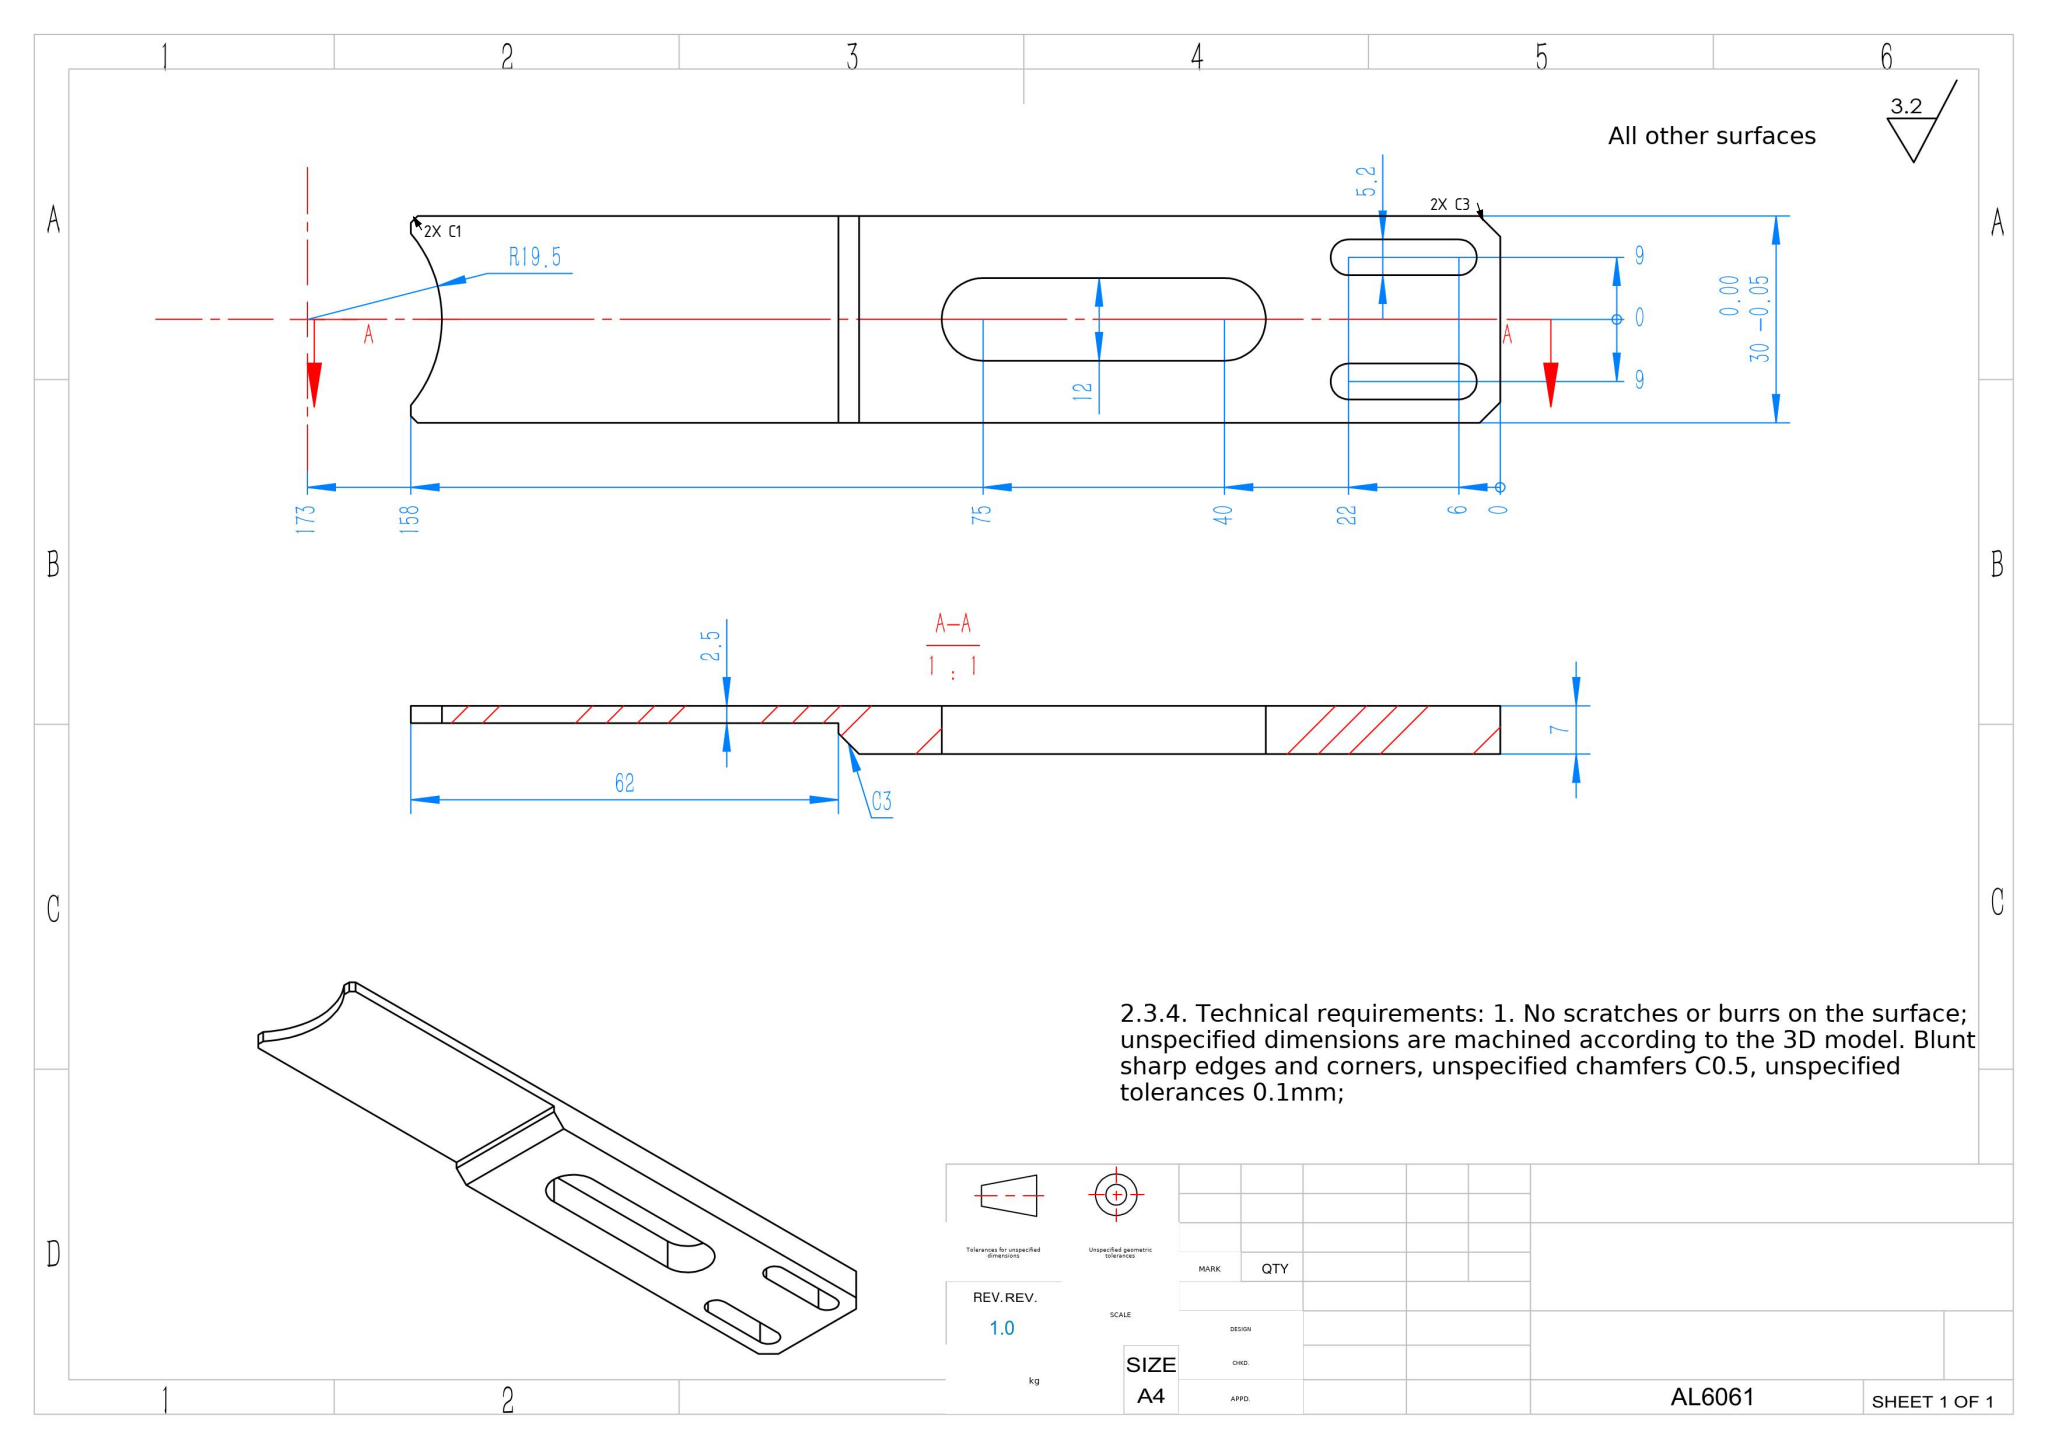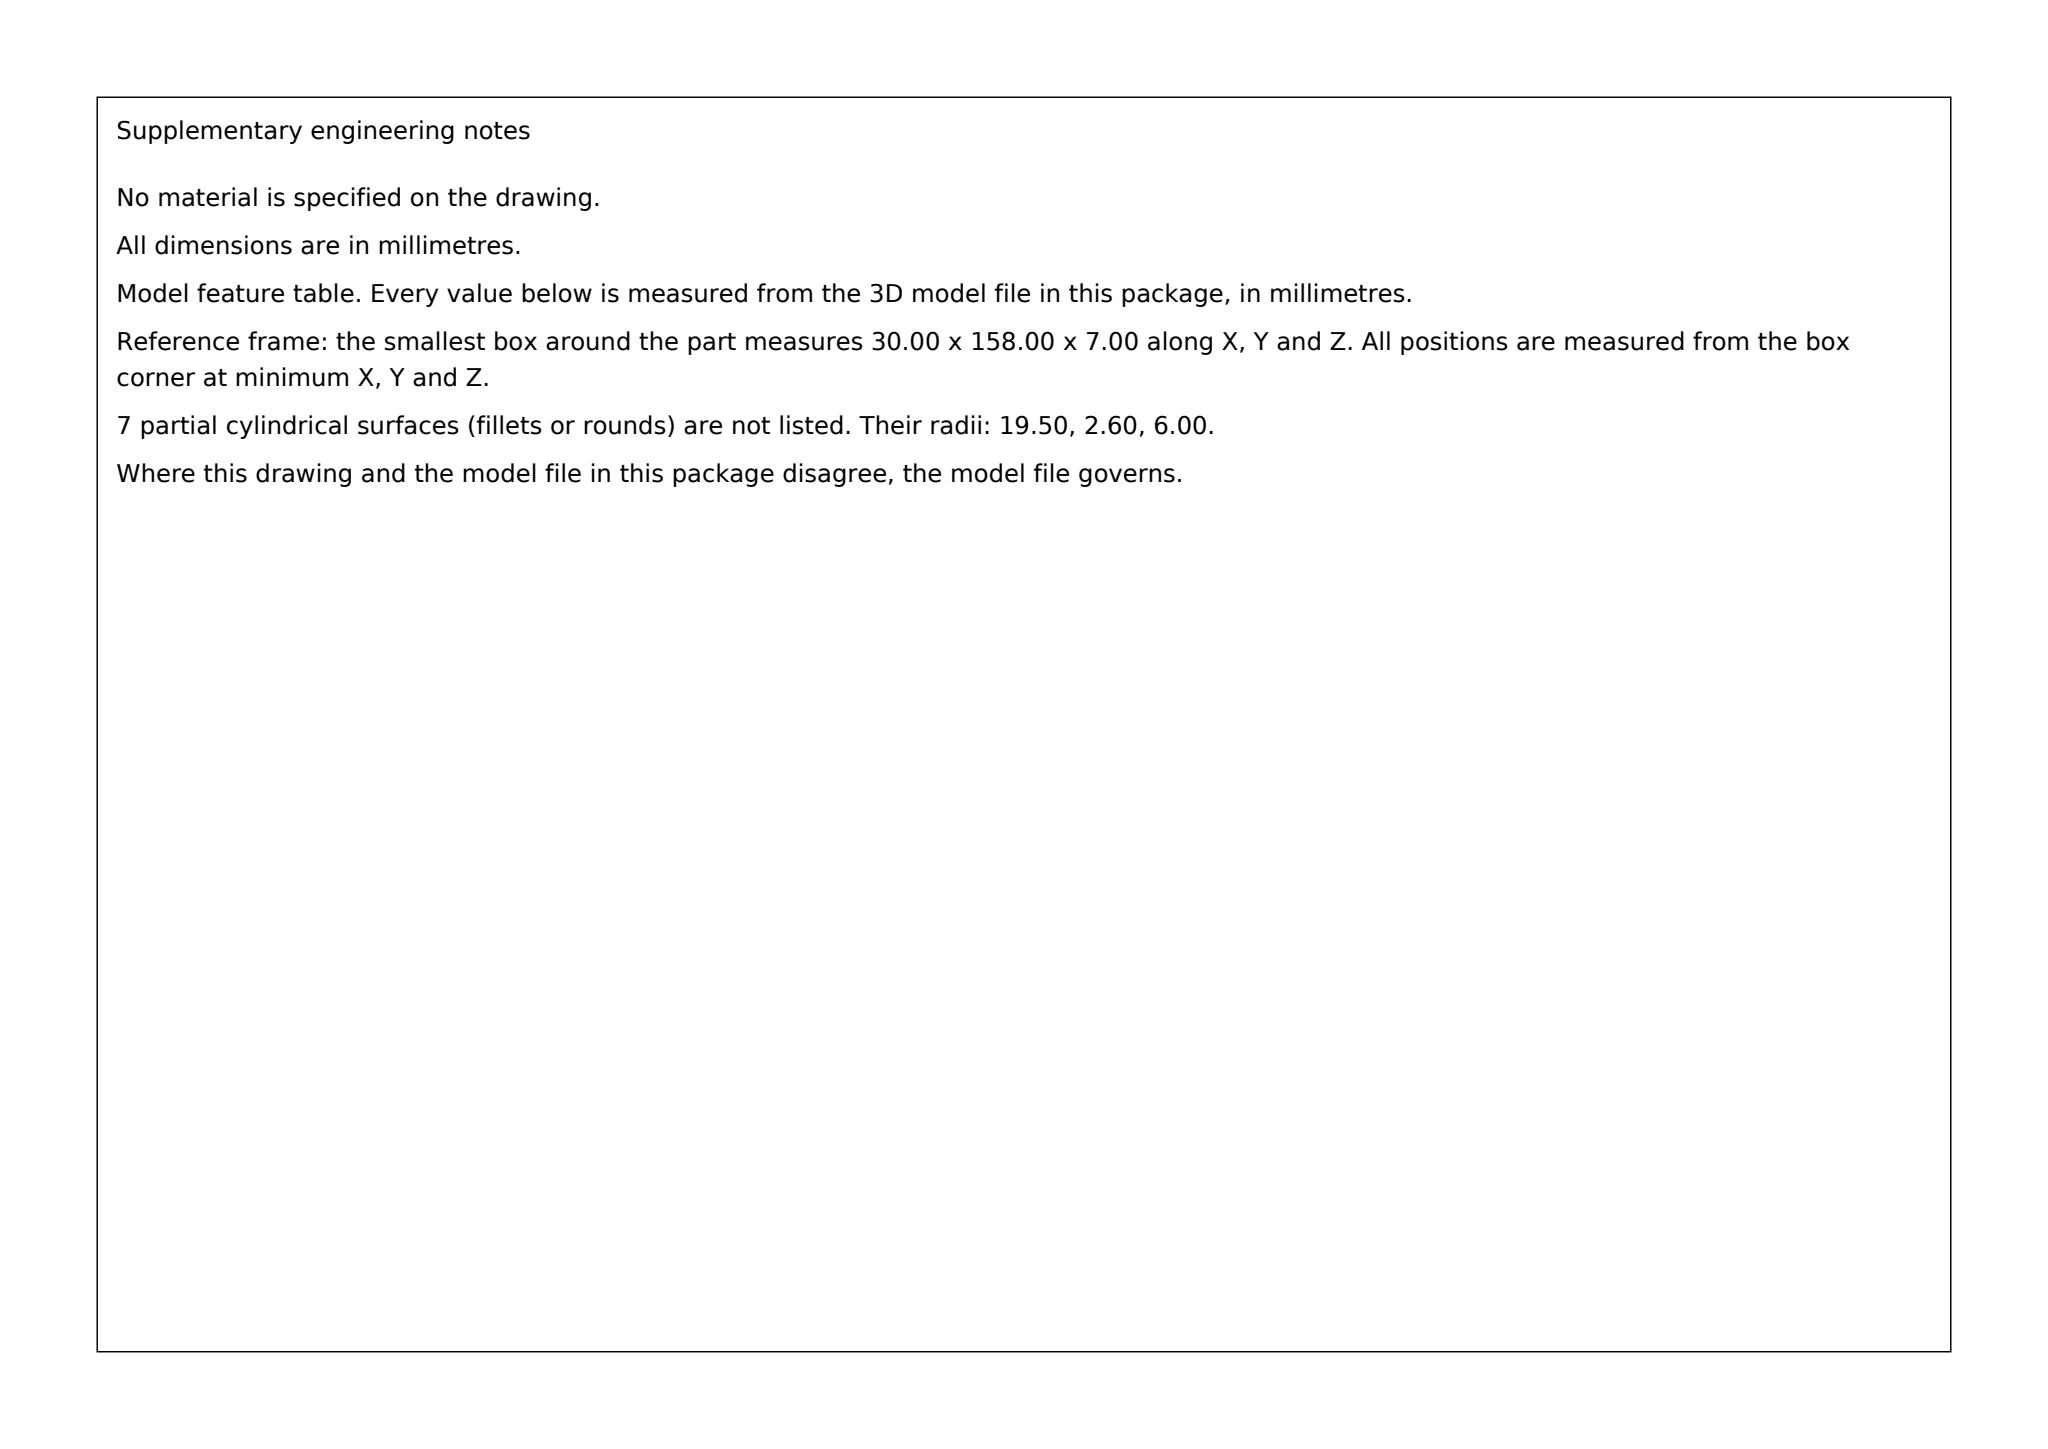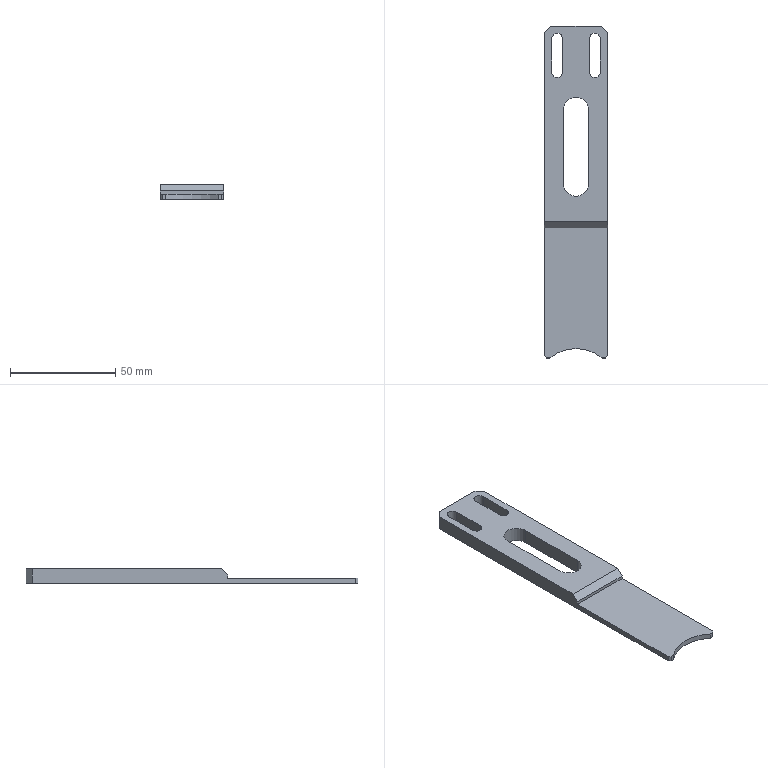Part | SolidWorks | mm | material AL6061 | 1 solid | 27 faces | box 30 x 158 x 7 mm | volume 19224 mm3 | plane 20 | cylinder 7 | commonest cylinder face diameters 5.2 x4 12 x2 39 x1
Drawing notes:
2X CHAMFER 3 X 45° ON THE TWO CORNERS OF THE 30 WIDE END FACE AT THE 0 DATUM END (158 FROM THE RADIUSED END), FULL 7 THICKNESS | from the solid: inclined_planes: two 45/45/90 faces, bbox_from [0,155,0] and [27,155,0], size [3,3,7]; y=158 end face extent x 3..27
2X CHAMFER 1 X 45° ON THE TWO CORNERS OF THE OPPOSITE (RADIUSED, 173 DATUM) END, WITHIN THE 2.5 THICK STEP | from the solid: inclined_planes: two 45/45/90 faces, bbox_from [0,0,0] and [29,0,0], size [1,1,2.5]
build123d program:
from build123d import *

# Parameters (mm, degrees)
SKETCH1_W               = 30
SKETCH1_H               = 158
BOSS_EXTRUDE1_DEPTH     = 1.25
SKETCH3_W               = 30
SKETCH3_H               = 96
BOSS_EXTRUDE2_DEPTH     = 4.5
CUT_EXTRUDE1_DEPTH      = 81.537
CUT_EXTRUDE1_DEPTH_BACK = 81.537
SKETCH2_R               = 19.5
CUT_EXTRUDE2_DEPTH      = 81.716
CHAMFER1_SIZE           = 3
CUT_EXTRUDE3_DEPTH      = 81.716
CHAMFER2_SIZE           = 3
CHAMFER4_SIZE           = 1


with BuildPart() as part:
    # Sketch1 → Boss-Extrude1 (new, symmetric)
    with BuildSketch(Plane.XY):
        Rectangle(SKETCH1_W, SKETCH1_H)
    extrude(amount=BOSS_EXTRUDE1_DEPTH, both=True)

    # Sketch3 → Boss-Extrude2 (add)
    with BuildSketch(Plane.XY.offset(1.25)):
        with Locations((0, 31)):
            Rectangle(SKETCH3_W, SKETCH3_H)
    extrude(amount=BOSS_EXTRUDE2_DEPTH)

    # Sketch2 → Cut-Extrude1 (cut, two sides: drawn at the far end of the back side and taken through both)
    with BuildSketch(Plane.XY.offset(1.25).offset(-CUT_EXTRUDE1_DEPTH_BACK)):
        with Locations((0, -94)):
            Circle(SKETCH2_R)
    extrude(amount=CUT_EXTRUDE1_DEPTH + CUT_EXTRUDE1_DEPTH_BACK, mode=Mode.SUBTRACT)

    # Sketch4 → Cut-Extrude2 (cut, through all)
    with BuildSketch(Plane.XY.offset(5.75)):
        with BuildLine():
            Line((-11.6, 57), (-11.6, 73))
            ThreePointArc((-11.6, 73), (-9, 75.6), (-6.4, 73))
            Line((-6.4, 73), (-6.4, 57))
            ThreePointArc((-6.4, 57), (-9, 54.4), (-11.6, 57))
        make_face()
        with BuildLine():
            Line((6.4, 57), (6.4, 73))
            ThreePointArc((6.4, 73), (9, 75.6), (11.6, 73))
            Line((11.6, 73), (11.6, 57))
            ThreePointArc((11.6, 57), (9, 54.4), (6.4, 57))
        make_face()
    extrude(amount=-CUT_EXTRUDE2_DEPTH, mode=Mode.SUBTRACT)

    # Chamfer1
    chamfer1_edges = [part.edges().sort_by_distance(p)[0] for p in [
        (0, -17, 5.75),
    ]]
    chamfer(chamfer1_edges, length=CHAMFER1_SIZE)

    # Sketch5 → Cut-Extrude3 (cut, through all)
    with BuildSketch(Plane.XY.offset(5.75)):
        with BuildLine():
            Line((-6, 4), (-6, 39))
            ThreePointArc((-6, 39), (0, 45), (6, 39))
            Line((6, 39), (6, 4))
            ThreePointArc((6, 4), (0, -2), (-6, 4))
        make_face()
    extrude(amount=-CUT_EXTRUDE3_DEPTH, mode=Mode.SUBTRACT)

    # Chamfer2
    chamfer2_edges = [part.edges().sort_by_distance(p)[0] for p in [
        (-15, 79, 2.25),
        (15, 79, 2.25),
    ]]
    chamfer(chamfer2_edges, length=CHAMFER2_SIZE)

    # Chamfer4
    chamfer4_edges = [part.edges().sort_by_distance(p)[0] for p in [
        (15, -79, 0),
        (-15, -79, 0),
    ]]
    chamfer(chamfer4_edges, length=CHAMFER4_SIZE)


solid = part.part
STEP:
#1=CARTESIAN_POINT('',(-14.,-79.,1.25));
#2=VERTEX_POINT('',#1);
#3=CARTESIAN_POINT('',(-12.46,-79.,1.25));
#4=VERTEX_POINT('',#3);
#5=CARTESIAN_POINT('',(-15.,-79.,1.25));
#6=DIRECTION('',(1.,0.,0.));
#7=VECTOR('',#6,1000.);
#8=LINE('',#5,#7);
#9=EDGE_CURVE('',#2,#4,#8,.T.);
#10=ORIENTED_EDGE('',*,*,#9,.F.);
#11=CARTESIAN_POINT('',(-14.,-79.,-1.25));
#12=VERTEX_POINT('',#11);
#13=CARTESIAN_POINT('',(-14.,-79.,1.25));
#14=DIRECTION('',(0.,0.,-1.));
#15=VECTOR('',#14,1000.);
#16=LINE('',#13,#15);
#17=EDGE_CURVE('',#2,#12,#16,.T.);
#18=ORIENTED_EDGE('',*,*,#17,.T.);
#19=CARTESIAN_POINT('',(-12.46,-79.,-1.25));
#20=VERTEX_POINT('',#19);
#21=CARTESIAN_POINT('',(-15.,-79.,-1.25));
#22=DIRECTION('',(1.,0.,0.));
#23=VECTOR('',#22,1000.);
#24=LINE('',#21,#23);
#25=EDGE_CURVE('',#12,#20,#24,.T.);
#26=ORIENTED_EDGE('',*,*,#25,.T.);
#27=CARTESIAN_POINT('',(-12.46,-79.,-1.25));
#28=DIRECTION('',(0.,0.,1.));
#29=VECTOR('',#28,1000.);
#30=LINE('',#27,#29);
#31=EDGE_CURVE('',#20,#4,#30,.T.);
#32=ORIENTED_EDGE('',*,*,#31,.T.);
#33=EDGE_LOOP('',(#10,#18,#26,#32));
#34=FACE_OUTER_BOUND('',#33,.T.);
#35=CARTESIAN_POINT('',(-15.,-79.,1.25));
#36=DIRECTION('',(0.,1.,0.));
#37=DIRECTION('',(0.,0.,1.));
#38=AXIS2_PLACEMENT_3D('',#35,#36,#37);
#39=PLANE('',#38);
#40=ADVANCED_FACE('',(#34),#39,.F.);
#41=CARTESIAN_POINT('',(-15.,-17.,1.25));
#42=VERTEX_POINT('',#41);
#43=CARTESIAN_POINT('',(-15.,-78.,1.25));
#44=VERTEX_POINT('',#43);
#45=CARTESIAN_POINT('',(-15.,-79.,1.25));
#46=DIRECTION('',(0.,-1.,0.));
#47=VECTOR('',#46,1000.);
#48=LINE('',#45,#47);
#49=EDGE_CURVE('',#42,#44,#48,.T.);
#50=ORIENTED_EDGE('',*,*,#49,.T.);
#51=CARTESIAN_POINT('',(-14.,-79.,1.25));
#52=DIRECTION('',(0.7071,-0.7071,0.));
#53=VECTOR('',#52,1000.);
#54=LINE('',#51,#53);
#55=EDGE_CURVE('',#44,#2,#54,.T.);
#56=ORIENTED_EDGE('',*,*,#55,.T.);
#57=ORIENTED_EDGE('',*,*,#9,.T.);
#58=CARTESIAN_POINT('',(12.46,-79.,1.25));
#59=VERTEX_POINT('',#58);
#60=CARTESIAN_POINT('',(0.,-94.,1.25));
#61=DIRECTION('',(0.,0.,-1.));
#62=DIRECTION('',(-1.,0.,0.));
#63=AXIS2_PLACEMENT_3D('',#60,#61,#62);
#64=CIRCLE('',#63,19.5);
#65=EDGE_CURVE('',#4,#59,#64,.T.);
#66=ORIENTED_EDGE('',*,*,#65,.T.);
#67=CARTESIAN_POINT('',(14.,-79.,1.25));
#68=VERTEX_POINT('',#67);
#69=CARTESIAN_POINT('',(-15.,-79.,1.25));
#70=DIRECTION('',(1.,0.,0.));
#71=VECTOR('',#70,1000.);
#72=LINE('',#69,#71);
#73=EDGE_CURVE('',#59,#68,#72,.T.);
#74=ORIENTED_EDGE('',*,*,#73,.T.);
#75=CARTESIAN_POINT('',(15.,-78.,1.25));
#76=VERTEX_POINT('',#75);
#77=CARTESIAN_POINT('',(15.,-78.,1.25));
#78=DIRECTION('',(0.7071,0.7071,0.));
#79=VECTOR('',#78,1000.);
#80=LINE('',#77,#79);
#81=EDGE_CURVE('',#68,#76,#80,.T.);
#82=ORIENTED_EDGE('',*,*,#81,.T.);
#83=CARTESIAN_POINT('',(15.,-17.,1.25));
#84=VERTEX_POINT('',#83);
#85=CARTESIAN_POINT('',(15.,-79.,1.25));
#86=DIRECTION('',(0.,1.,0.));
#87=VECTOR('',#86,1000.);
#88=LINE('',#85,#87);
#89=EDGE_CURVE('',#76,#84,#88,.T.);
#90=ORIENTED_EDGE('',*,*,#89,.T.);
#91=CARTESIAN_POINT('',(-15.,-17.,1.25));
#92=DIRECTION('',(1.,0.,0.));
#93=VECTOR('',#92,1000.);
#94=LINE('',#91,#93);
#95=EDGE_CURVE('',#42,#84,#94,.T.);
#96=ORIENTED_EDGE('',*,*,#95,.F.);
#97=EDGE_LOOP('',(#50,#56,#57,#66,#74,#82,#90,#96));
#98=FACE_OUTER_BOUND('',#97,.T.);
#99=CARTESIAN_POINT('',(0.,0.,1.25));
#100=DIRECTION('',(0.,0.,-1.));
#101=DIRECTION('',(-1.,0.,0.));
#102=AXIS2_PLACEMENT_3D('',#99,#100,#101);
#103=PLANE('',#102);
#104=ADVANCED_FACE('',(#98),#103,.F.);
#105=ORIENTED_EDGE('',*,*,#89,.F.);
#106=CARTESIAN_POINT('',(15.,-78.,-1.25));
#107=VERTEX_POINT('',#106);
#108=CARTESIAN_POINT('',(15.,-78.,1.25));
#109=DIRECTION('',(0.,0.,-1.));
#110=VECTOR('',#109,1000.);
#111=LINE('',#108,#110);
#112=EDGE_CURVE('',#76,#107,#111,.T.);
#113=ORIENTED_EDGE('',*,*,#112,.T.);
#114=CARTESIAN_POINT('',(15.,76.,-1.25));
#115=VERTEX_POINT('',#114);
#116=CARTESIAN_POINT('',(15.,-79.,-1.25));
#117=DIRECTION('',(0.,1.,0.));
#118=VECTOR('',#117,1000.);
#119=LINE('',#116,#118);
#120=EDGE_CURVE('',#107,#115,#119,.T.);
#121=ORIENTED_EDGE('',*,*,#120,.T.);
#122=CARTESIAN_POINT('',(15.,76.,5.75));
#123=VERTEX_POINT('',#122);
#124=CARTESIAN_POINT('',(15.,76.,1.25));
#125=DIRECTION('',(0.,0.,1.));
#126=VECTOR('',#125,1000.);
#127=LINE('',#124,#126);
#128=EDGE_CURVE('',#115,#123,#127,.T.);
#129=ORIENTED_EDGE('',*,*,#128,.T.);
#130=CARTESIAN_POINT('',(15.,-14.,5.75));
#131=VERTEX_POINT('',#130);
#132=CARTESIAN_POINT('',(15.,79.,5.75));
#133=DIRECTION('',(-0.,1.,0.));
#134=VECTOR('',#133,1000.);
#135=LINE('',#132,#134);
#136=EDGE_CURVE('',#131,#123,#135,.T.);
#137=ORIENTED_EDGE('',*,*,#136,.F.);
#138=CARTESIAN_POINT('',(15.,-17.,2.75));
#139=VERTEX_POINT('',#138);
#140=CARTESIAN_POINT('',(15.,-14.,5.75));
#141=DIRECTION('',(0.,-0.7071,-0.7071));
#142=VECTOR('',#141,1000.);
#143=LINE('',#140,#142);
#144=EDGE_CURVE('',#131,#139,#143,.T.);
#145=ORIENTED_EDGE('',*,*,#144,.T.);
#146=CARTESIAN_POINT('',(15.,-17.,5.75));
#147=DIRECTION('',(0.,0.,-1.));
#148=VECTOR('',#147,1000.);
#149=LINE('',#146,#148);
#150=EDGE_CURVE('',#139,#84,#149,.T.);
#151=ORIENTED_EDGE('',*,*,#150,.T.);
#152=EDGE_LOOP('',(#105,#113,#121,#129,#137,#145,#151));
#153=FACE_OUTER_BOUND('',#152,.T.);
#154=CARTESIAN_POINT('',(15.,-79.,1.25));
#155=DIRECTION('',(-1.,0.,0.));
#156=DIRECTION('',(0.,0.,1.));
#157=AXIS2_PLACEMENT_3D('',#154,#155,#156);
#158=PLANE('',#157);
#159=ADVANCED_FACE('',(#153),#158,.F.);
#160=CARTESIAN_POINT('',(12.,79.,-1.25));
#161=VERTEX_POINT('',#160);
#162=CARTESIAN_POINT('',(-12.,79.,-1.25));
#163=VERTEX_POINT('',#162);
#164=CARTESIAN_POINT('',(-15.,79.,-1.25));
#165=DIRECTION('',(-1.,0.,0.));
#166=VECTOR('',#165,1000.);
#167=LINE('',#164,#166);
#168=EDGE_CURVE('',#161,#163,#167,.T.);
#169=ORIENTED_EDGE('',*,*,#168,.T.);
#170=CARTESIAN_POINT('',(-12.,79.,5.75));
#171=VERTEX_POINT('',#170);
#172=CARTESIAN_POINT('',(-12.,79.,1.25));
#173=DIRECTION('',(0.,0.,1.));
#174=VECTOR('',#173,1000.);
#175=LINE('',#172,#174);
#176=EDGE_CURVE('',#163,#171,#175,.T.);
#177=ORIENTED_EDGE('',*,*,#176,.T.);
#178=CARTESIAN_POINT('',(12.,79.,5.75));
#179=VERTEX_POINT('',#178);
#180=CARTESIAN_POINT('',(-15.,79.,5.75));
#181=DIRECTION('',(-1.,0.,0.));
#182=VECTOR('',#181,1000.);
#183=LINE('',#180,#182);
#184=EDGE_CURVE('',#179,#171,#183,.T.);
#185=ORIENTED_EDGE('',*,*,#184,.F.);
#186=CARTESIAN_POINT('',(12.,79.,1.25));
#187=DIRECTION('',(0.,0.,-1.));
#188=VECTOR('',#187,1000.);
#189=LINE('',#186,#188);
#190=EDGE_CURVE('',#179,#161,#189,.T.);
#191=ORIENTED_EDGE('',*,*,#190,.T.);
#192=EDGE_LOOP('',(#169,#177,#185,#191));
#193=FACE_OUTER_BOUND('',#192,.T.);
#194=CARTESIAN_POINT('',(-15.,79.,1.25));
#195=DIRECTION('',(0.,-1.,0.));
#196=DIRECTION('',(0.,0.,-1.));
#197=AXIS2_PLACEMENT_3D('',#194,#195,#196);
#198=PLANE('',#197);
#199=ADVANCED_FACE('',(#193),#198,.F.);
#200=CARTESIAN_POINT('',(-15.,76.,-1.25));
#201=VERTEX_POINT('',#200);
#202=CARTESIAN_POINT('',(-15.,-78.,-1.25));
#203=VERTEX_POINT('',#202);
#204=CARTESIAN_POINT('',(-15.,-79.,-1.25));
#205=DIRECTION('',(0.,-1.,0.));
#206=VECTOR('',#205,1000.);
#207=LINE('',#204,#206);
#208=EDGE_CURVE('',#201,#203,#207,.T.);
#209=ORIENTED_EDGE('',*,*,#208,.T.);
#210=CARTESIAN_POINT('',(-15.,-78.,1.25));
#211=DIRECTION('',(0.,0.,1.));
#212=VECTOR('',#211,1000.);
#213=LINE('',#210,#212);
#214=EDGE_CURVE('',#203,#44,#213,.T.);
#215=ORIENTED_EDGE('',*,*,#214,.T.);
#216=ORIENTED_EDGE('',*,*,#49,.F.);
#217=CARTESIAN_POINT('',(-15.,-17.,2.75));
#218=VERTEX_POINT('',#217);
#219=CARTESIAN_POINT('',(-15.,-17.,5.75));
#220=DIRECTION('',(0.,0.,-1.));
#221=VECTOR('',#220,1000.);
#222=LINE('',#219,#221);
#223=EDGE_CURVE('',#218,#42,#222,.T.);
#224=ORIENTED_EDGE('',*,*,#223,.F.);
#225=CARTESIAN_POINT('',(-15.,-14.,5.75));
#226=VERTEX_POINT('',#225);
#227=CARTESIAN_POINT('',(-15.,-14.,5.75));
#228=DIRECTION('',(0.,0.7071,0.7071));
#229=VECTOR('',#228,1000.);
#230=LINE('',#227,#229);
#231=EDGE_CURVE('',#218,#226,#230,.T.);
#232=ORIENTED_EDGE('',*,*,#231,.T.);
#233=CARTESIAN_POINT('',(-15.,76.,5.75));
#234=VERTEX_POINT('',#233);
#235=CARTESIAN_POINT('',(-15.,79.,5.75));
#236=DIRECTION('',(0.,-1.,0.));
#237=VECTOR('',#236,1000.);
#238=LINE('',#235,#237);
#239=EDGE_CURVE('',#234,#226,#238,.T.);
#240=ORIENTED_EDGE('',*,*,#239,.F.);
#241=CARTESIAN_POINT('',(-15.,76.,1.25));
#242=DIRECTION('',(0.,0.,-1.));
#243=VECTOR('',#242,1000.);
#244=LINE('',#241,#243);
#245=EDGE_CURVE('',#234,#201,#244,.T.);
#246=ORIENTED_EDGE('',*,*,#245,.T.);
#247=EDGE_LOOP('',(#209,#215,#216,#224,#232,#240,#246));
#248=FACE_OUTER_BOUND('',#247,.T.);
#249=CARTESIAN_POINT('',(-15.,-79.,1.25));
#250=DIRECTION('',(1.,0.,0.));
#251=DIRECTION('',(0.,0.,-1.));
#252=AXIS2_PLACEMENT_3D('',#249,#250,#251);
#253=PLANE('',#252);
#254=ADVANCED_FACE('',(#248),#253,.F.);
#255=CARTESIAN_POINT('',(12.46,-79.,-1.25));
#256=VERTEX_POINT('',#255);
#257=CARTESIAN_POINT('',(14.,-79.,-1.25));
#258=VERTEX_POINT('',#257);
#259=CARTESIAN_POINT('',(-15.,-79.,-1.25));
#260=DIRECTION('',(1.,0.,0.));
#261=VECTOR('',#260,1000.);
#262=LINE('',#259,#261);
#263=EDGE_CURVE('',#256,#258,#262,.T.);
#264=ORIENTED_EDGE('',*,*,#263,.T.);
#265=CARTESIAN_POINT('',(14.,-79.,1.25));
#266=DIRECTION('',(0.,0.,1.));
#267=VECTOR('',#266,1000.);
#268=LINE('',#265,#267);
#269=EDGE_CURVE('',#258,#68,#268,.T.);
#270=ORIENTED_EDGE('',*,*,#269,.T.);
#271=ORIENTED_EDGE('',*,*,#73,.F.);
#272=CARTESIAN_POINT('',(12.46,-79.,-1.25));
#273=DIRECTION('',(0.,0.,-1.));
#274=VECTOR('',#273,1000.);
#275=LINE('',#272,#274);
#276=EDGE_CURVE('',#59,#256,#275,.T.);
#277=ORIENTED_EDGE('',*,*,#276,.T.);
#278=EDGE_LOOP('',(#264,#270,#271,#277));
#279=FACE_OUTER_BOUND('',#278,.T.);
#280=CARTESIAN_POINT('',(-15.,-79.,1.25));
#281=DIRECTION('',(0.,1.,0.));
#282=DIRECTION('',(0.,0.,1.));
#283=AXIS2_PLACEMENT_3D('',#280,#281,#282);
#284=PLANE('',#283);
#285=ADVANCED_FACE('',(#279),#284,.F.);
#286=CARTESIAN_POINT('',(-6.,4.,-1.25));
#287=VERTEX_POINT('',#286);
#288=CARTESIAN_POINT('',(6.,4.,-1.25));
#289=VERTEX_POINT('',#288);
#290=CARTESIAN_POINT('',(0.,4.,-1.25));
#291=DIRECTION('',(0.,0.,1.));
#292=DIRECTION('',(1.,0.,0.));
#293=AXIS2_PLACEMENT_3D('',#290,#291,#292);
#294=CIRCLE('',#293,6.);
#295=EDGE_CURVE('',#287,#289,#294,.T.);
#296=ORIENTED_EDGE('',*,*,#295,.T.);
#297=CARTESIAN_POINT('',(6.,39.,-1.25));
#298=VERTEX_POINT('',#297);
#299=CARTESIAN_POINT('',(6.,4.,-1.25));
#300=DIRECTION('',(-0.,1.,0.));
#301=VECTOR('',#300,1000.);
#302=LINE('',#299,#301);
#303=EDGE_CURVE('',#289,#298,#302,.T.);
#304=ORIENTED_EDGE('',*,*,#303,.T.);
#305=CARTESIAN_POINT('',(-6.,39.,-1.25));
#306=VERTEX_POINT('',#305);
#307=CARTESIAN_POINT('',(0.,39.,-1.25));
#308=DIRECTION('',(0.,0.,1.));
#309=DIRECTION('',(1.,0.,0.));
#310=AXIS2_PLACEMENT_3D('',#307,#308,#309);
#311=CIRCLE('',#310,6.);
#312=EDGE_CURVE('',#298,#306,#311,.T.);
#313=ORIENTED_EDGE('',*,*,#312,.T.);
#314=CARTESIAN_POINT('',(-6.,4.,-1.25));
#315=DIRECTION('',(-0.,-1.,0.));
#316=VECTOR('',#315,1000.);
#317=LINE('',#314,#316);
#318=EDGE_CURVE('',#306,#287,#317,.T.);
#319=ORIENTED_EDGE('',*,*,#318,.T.);
#320=EDGE_LOOP('',(#296,#304,#313,#319));
#321=FACE_BOUND('',#320,.T.);
#322=CARTESIAN_POINT('',(-11.6,57.,-1.25));
#323=VERTEX_POINT('',#322);
#324=CARTESIAN_POINT('',(-6.4,57.,-1.25));
#325=VERTEX_POINT('',#324);
#326=CARTESIAN_POINT('',(-9.,57.,-1.25));
#327=DIRECTION('',(0.,0.,1.));
#328=DIRECTION('',(1.,0.,0.));
#329=AXIS2_PLACEMENT_3D('',#326,#327,#328);
#330=CIRCLE('',#329,2.6);
#331=EDGE_CURVE('',#323,#325,#330,.T.);
#332=ORIENTED_EDGE('',*,*,#331,.T.);
#333=CARTESIAN_POINT('',(-6.4,73.,-1.25));
#334=VERTEX_POINT('',#333);
#335=CARTESIAN_POINT('',(-6.4,57.,-1.25));
#336=DIRECTION('',(-0.,1.,0.));
#337=VECTOR('',#336,1000.);
#338=LINE('',#335,#337);
#339=EDGE_CURVE('',#325,#334,#338,.T.);
#340=ORIENTED_EDGE('',*,*,#339,.T.);
#341=CARTESIAN_POINT('',(-11.6,73.,-1.25));
#342=VERTEX_POINT('',#341);
#343=CARTESIAN_POINT('',(-9.,73.,-1.25));
#344=DIRECTION('',(0.,0.,1.));
#345=DIRECTION('',(1.,0.,0.));
#346=AXIS2_PLACEMENT_3D('',#343,#344,#345);
#347=CIRCLE('',#346,2.6);
#348=EDGE_CURVE('',#334,#342,#347,.T.);
#349=ORIENTED_EDGE('',*,*,#348,.T.);
#350=CARTESIAN_POINT('',(-11.6,57.,-1.25));
#351=DIRECTION('',(0.,-1.,0.));
#352=VECTOR('',#351,1000.);
#353=LINE('',#350,#352);
#354=EDGE_CURVE('',#342,#323,#353,.T.);
#355=ORIENTED_EDGE('',*,*,#354,.T.);
#356=EDGE_LOOP('',(#332,#340,#349,#355));
#357=FACE_BOUND('',#356,.T.);
#358=CARTESIAN_POINT('',(6.4,57.,-1.25));
#359=VERTEX_POINT('',#358);
#360=CARTESIAN_POINT('',(11.6,57.,-1.25));
#361=VERTEX_POINT('',#360);
#362=CARTESIAN_POINT('',(9.,57.,-1.25));
#363=DIRECTION('',(0.,0.,1.));
#364=DIRECTION('',(1.,0.,0.));
#365=AXIS2_PLACEMENT_3D('',#362,#363,#364);
#366=CIRCLE('',#365,2.6);
#367=EDGE_CURVE('',#359,#361,#366,.T.);
#368=ORIENTED_EDGE('',*,*,#367,.T.);
#369=CARTESIAN_POINT('',(11.6,73.,-1.25));
#370=VERTEX_POINT('',#369);
#371=CARTESIAN_POINT('',(11.6,57.,-1.25));
#372=DIRECTION('',(-0.,1.,0.));
#373=VECTOR('',#372,1000.);
#374=LINE('',#371,#373);
#375=EDGE_CURVE('',#361,#370,#374,.T.);
#376=ORIENTED_EDGE('',*,*,#375,.T.);
#377=CARTESIAN_POINT('',(6.4,73.,-1.25));
#378=VERTEX_POINT('',#377);
#379=CARTESIAN_POINT('',(9.,73.,-1.25));
#380=DIRECTION('',(0.,0.,1.));
#381=DIRECTION('',(1.,0.,0.));
#382=AXIS2_PLACEMENT_3D('',#379,#380,#381);
#383=CIRCLE('',#382,2.6);
#384=EDGE_CURVE('',#370,#378,#383,.T.);
#385=ORIENTED_EDGE('',*,*,#384,.T.);
#386=CARTESIAN_POINT('',(6.4,57.,-1.25));
#387=DIRECTION('',(0.,-1.,0.));
#388=VECTOR('',#387,1000.);
#389=LINE('',#386,#388);
#390=EDGE_CURVE('',#378,#359,#389,.T.);
#391=ORIENTED_EDGE('',*,*,#390,.T.);
#392=EDGE_LOOP('',(#368,#376,#385,#391));
#393=FACE_BOUND('',#392,.T.);
#394=ORIENTED_EDGE('',*,*,#25,.F.);
#395=CARTESIAN_POINT('',(-46.5,-46.5,-1.25));
#396=DIRECTION('',(-0.7071,0.7071,0.));
#397=VECTOR('',#396,1000.);
#398=LINE('',#395,#397);
#399=EDGE_CURVE('',#12,#203,#398,.T.);
#400=ORIENTED_EDGE('',*,*,#399,.T.);
#401=ORIENTED_EDGE('',*,*,#208,.F.);
#402=CARTESIAN_POINT('',(-45.5,45.5,-1.25));
#403=DIRECTION('',(0.7071,0.7071,0.));
#404=VECTOR('',#403,1000.);
#405=LINE('',#402,#404);
#406=EDGE_CURVE('',#201,#163,#405,.T.);
#407=ORIENTED_EDGE('',*,*,#406,.T.);
#408=ORIENTED_EDGE('',*,*,#168,.F.);
#409=CARTESIAN_POINT('',(45.5,45.5,-1.25));
#410=DIRECTION('',(0.7071,-0.7071,0.));
#411=VECTOR('',#410,1000.);
#412=LINE('',#409,#411);
#413=EDGE_CURVE('',#161,#115,#412,.T.);
#414=ORIENTED_EDGE('',*,*,#413,.T.);
#415=ORIENTED_EDGE('',*,*,#120,.F.);
#416=CARTESIAN_POINT('',(46.5,-46.5,-1.25));
#417=DIRECTION('',(-0.7071,-0.7071,0.));
#418=VECTOR('',#417,1000.);
#419=LINE('',#416,#418);
#420=EDGE_CURVE('',#107,#258,#419,.T.);
#421=ORIENTED_EDGE('',*,*,#420,.T.);
#422=ORIENTED_EDGE('',*,*,#263,.F.);
#423=CARTESIAN_POINT('',(0.,-94.,-1.25));
#424=DIRECTION('',(0.,0.,1.));
#425=DIRECTION('',(1.,0.,0.));
#426=AXIS2_PLACEMENT_3D('',#423,#424,#425);
#427=CIRCLE('',#426,19.5);
#428=EDGE_CURVE('',#256,#20,#427,.T.);
#429=ORIENTED_EDGE('',*,*,#428,.T.);
#430=EDGE_LOOP('',(#394,#400,#401,#407,#408,#414,#415,#421,#422,#429));
#431=FACE_OUTER_BOUND('',#430,.T.);
#432=CARTESIAN_POINT('',(0.,0.,-1.25));
#433=DIRECTION('',(0.,0.,-1.));
#434=DIRECTION('',(-1.,0.,0.));
#435=AXIS2_PLACEMENT_3D('',#432,#433,#434);
#436=PLANE('',#435);
#437=ADVANCED_FACE('',(#321,#357,#393,#431),#436,.T.);
#438=ORIENTED_EDGE('',*,*,#150,.F.);
#439=CARTESIAN_POINT('',(-15.,-17.,2.75));
#440=DIRECTION('',(-1.,0.,0.));
#441=VECTOR('',#440,1000.);
#442=LINE('',#439,#441);
#443=EDGE_CURVE('',#139,#218,#442,.T.);
#444=ORIENTED_EDGE('',*,*,#443,.T.);
#445=ORIENTED_EDGE('',*,*,#223,.T.);
#446=ORIENTED_EDGE('',*,*,#95,.T.);
#447=EDGE_LOOP('',(#438,#444,#445,#446));
#448=FACE_OUTER_BOUND('',#447,.T.);
#449=CARTESIAN_POINT('',(-15.,-17.,5.75));
#450=DIRECTION('',(0.,1.,0.));
#451=DIRECTION('',(0.,0.,1.));
#452=AXIS2_PLACEMENT_3D('',#449,#450,#451);
#453=PLANE('',#452);
#454=ADVANCED_FACE('',(#448),#453,.F.);
#455=CARTESIAN_POINT('',(-6.,4.,5.75));
#456=VERTEX_POINT('',#455);
#457=CARTESIAN_POINT('',(6.,4.,5.75));
#458=VERTEX_POINT('',#457);
#459=CARTESIAN_POINT('',(0.,4.,5.75));
#460=DIRECTION('',(0.,0.,1.));
#461=DIRECTION('',(1.,0.,0.));
#462=AXIS2_PLACEMENT_3D('',#459,#460,#461);
#463=CIRCLE('',#462,6.);
#464=EDGE_CURVE('',#456,#458,#463,.T.);
#465=ORIENTED_EDGE('',*,*,#464,.F.);
#466=CARTESIAN_POINT('',(-6.,39.,5.75));
#467=VERTEX_POINT('',#466);
#468=CARTESIAN_POINT('',(-6.,4.,5.75));
#469=DIRECTION('',(-0.,-1.,0.));
#470=VECTOR('',#469,1000.);
#471=LINE('',#468,#470);
#472=EDGE_CURVE('',#467,#456,#471,.T.);
#473=ORIENTED_EDGE('',*,*,#472,.F.);
#474=CARTESIAN_POINT('',(6.,39.,5.75));
#475=VERTEX_POINT('',#474);
#476=CARTESIAN_POINT('',(0.,39.,5.75));
#477=DIRECTION('',(0.,0.,1.));
#478=DIRECTION('',(1.,0.,0.));
#479=AXIS2_PLACEMENT_3D('',#476,#477,#478);
#480=CIRCLE('',#479,6.);
#481=EDGE_CURVE('',#475,#467,#480,.T.);
#482=ORIENTED_EDGE('',*,*,#481,.F.);
#483=CARTESIAN_POINT('',(6.,4.,5.75));
#484=DIRECTION('',(-0.,1.,0.));
#485=VECTOR('',#484,1000.);
#486=LINE('',#483,#485);
#487=EDGE_CURVE('',#458,#475,#486,.T.);
#488=ORIENTED_EDGE('',*,*,#487,.F.);
#489=EDGE_LOOP('',(#465,#473,#482,#488));
#490=FACE_BOUND('',#489,.T.);
#491=CARTESIAN_POINT('',(-11.6,57.,5.75));
#492=VERTEX_POINT('',#491);
#493=CARTESIAN_POINT('',(-6.4,57.,5.75));
#494=VERTEX_POINT('',#493);
#495=CARTESIAN_POINT('',(-9.,57.,5.75));
#496=DIRECTION('',(0.,0.,1.));
#497=DIRECTION('',(1.,0.,0.));
#498=AXIS2_PLACEMENT_3D('',#495,#496,#497);
#499=CIRCLE('',#498,2.6);
#500=EDGE_CURVE('',#492,#494,#499,.T.);
#501=ORIENTED_EDGE('',*,*,#500,.F.);
#502=CARTESIAN_POINT('',(-11.6,73.,5.75));
#503=VERTEX_POINT('',#502);
#504=CARTESIAN_POINT('',(-11.6,57.,5.75));
#505=DIRECTION('',(0.,-1.,0.));
#506=VECTOR('',#505,1000.);
#507=LINE('',#504,#506);
#508=EDGE_CURVE('',#503,#492,#507,.T.);
#509=ORIENTED_EDGE('',*,*,#508,.F.);
#510=CARTESIAN_POINT('',(-6.4,73.,5.75));
#511=VERTEX_POINT('',#510);
#512=CARTESIAN_POINT('',(-9.,73.,5.75));
#513=DIRECTION('',(0.,0.,1.));
#514=DIRECTION('',(1.,0.,0.));
#515=AXIS2_PLACEMENT_3D('',#512,#513,#514);
#516=CIRCLE('',#515,2.6);
#517=EDGE_CURVE('',#511,#503,#516,.T.);
#518=ORIENTED_EDGE('',*,*,#517,.F.);
#519=CARTESIAN_POINT('',(-6.4,57.,5.75));
#520=DIRECTION('',(-0.,1.,0.));
#521=VECTOR('',#520,1000.);
#522=LINE('',#519,#521);
#523=EDGE_CURVE('',#494,#511,#522,.T.);
#524=ORIENTED_EDGE('',*,*,#523,.F.);
#525=EDGE_LOOP('',(#501,#509,#518,#524));
#526=FACE_BOUND('',#525,.T.);
#527=CARTESIAN_POINT('',(6.4,57.,5.75));
#528=VERTEX_POINT('',#527);
#529=CARTESIAN_POINT('',(11.6,57.,5.75));
#530=VERTEX_POINT('',#529);
#531=CARTESIAN_POINT('',(9.,57.,5.75));
#532=DIRECTION('',(0.,0.,1.));
#533=DIRECTION('',(1.,0.,0.));
#534=AXIS2_PLACEMENT_3D('',#531,#532,#533);
#535=CIRCLE('',#534,2.6);
#536=EDGE_CURVE('',#528,#530,#535,.T.);
#537=ORIENTED_EDGE('',*,*,#536,.F.);
#538=CARTESIAN_POINT('',(6.4,73.,5.75));
#539=VERTEX_POINT('',#538);
#540=CARTESIAN_POINT('',(6.4,57.,5.75));
#541=DIRECTION('',(0.,-1.,0.));
#542=VECTOR('',#541,1000.);
#543=LINE('',#540,#542);
#544=EDGE_CURVE('',#539,#528,#543,.T.);
#545=ORIENTED_EDGE('',*,*,#544,.F.);
#546=CARTESIAN_POINT('',(11.6,73.,5.75));
#547=VERTEX_POINT('',#546);
#548=CARTESIAN_POINT('',(9.,73.,5.75));
#549=DIRECTION('',(0.,0.,1.));
#550=DIRECTION('',(1.,0.,0.));
#551=AXIS2_PLACEMENT_3D('',#548,#549,#550);
#552=CIRCLE('',#551,2.6);
#553=EDGE_CURVE('',#547,#539,#552,.T.);
#554=ORIENTED_EDGE('',*,*,#553,.F.);
#555=CARTESIAN_POINT('',(11.6,57.,5.75));
#556=DIRECTION('',(-0.,1.,0.));
#557=VECTOR('',#556,1000.);
#558=LINE('',#555,#557);
#559=EDGE_CURVE('',#530,#547,#558,.T.);
#560=ORIENTED_EDGE('',*,*,#559,.F.);
#561=EDGE_LOOP('',(#537,#545,#554,#560));
#562=FACE_BOUND('',#561,.T.);
#563=ORIENTED_EDGE('',*,*,#184,.T.);
#564=CARTESIAN_POINT('',(-45.5,45.5,5.75));
#565=DIRECTION('',(-0.7071,-0.7071,0.));
#566=VECTOR('',#565,1000.);
#567=LINE('',#564,#566);
#568=EDGE_CURVE('',#171,#234,#567,.T.);
#569=ORIENTED_EDGE('',*,*,#568,.T.);
#570=ORIENTED_EDGE('',*,*,#239,.T.);
#571=CARTESIAN_POINT('',(15.,-14.,5.75));
#572=DIRECTION('',(1.,0.,0.));
#573=VECTOR('',#572,1000.);
#574=LINE('',#571,#573);
#575=EDGE_CURVE('',#226,#131,#574,.T.);
#576=ORIENTED_EDGE('',*,*,#575,.T.);
#577=ORIENTED_EDGE('',*,*,#136,.T.);
#578=CARTESIAN_POINT('',(45.5,45.5,5.75));
#579=DIRECTION('',(-0.7071,0.7071,0.));
#580=VECTOR('',#579,1000.);
#581=LINE('',#578,#580);
#582=EDGE_CURVE('',#123,#179,#581,.T.);
#583=ORIENTED_EDGE('',*,*,#582,.T.);
#584=EDGE_LOOP('',(#563,#569,#570,#576,#577,#583));
#585=FACE_OUTER_BOUND('',#584,.T.);
#586=CARTESIAN_POINT('',(0.,0.,5.75));
#587=DIRECTION('',(0.,0.,1.));
#588=DIRECTION('',(1.,0.,0.));
#589=AXIS2_PLACEMENT_3D('',#586,#587,#588);
#590=PLANE('',#589);
#591=ADVANCED_FACE('',(#490,#526,#562,#585),#590,.T.);
#592=ORIENTED_EDGE('',*,*,#428,.F.);
#593=ORIENTED_EDGE('',*,*,#276,.F.);
#594=ORIENTED_EDGE('',*,*,#65,.F.);
#595=ORIENTED_EDGE('',*,*,#31,.F.);
#596=EDGE_LOOP('',(#592,#593,#594,#595));
#597=FACE_OUTER_BOUND('',#596,.T.);
#598=CARTESIAN_POINT('',(0.,-94.,-1.25));
#599=DIRECTION('',(0.,0.,1.));
#600=DIRECTION('',(1.,0.,0.));
#601=AXIS2_PLACEMENT_3D('',#598,#599,#600);
#602=CYLINDRICAL_SURFACE('',#601,19.5);
#603=ADVANCED_FACE('',(#597),#602,.F.);
#604=ORIENTED_EDGE('',*,*,#536,.T.);
#605=CARTESIAN_POINT('',(11.6,57.,-1.25));
#606=DIRECTION('',(0.,0.,1.));
#607=VECTOR('',#606,1000.);
#608=LINE('',#605,#607);
#609=EDGE_CURVE('',#361,#530,#608,.T.);
#610=ORIENTED_EDGE('',*,*,#609,.F.);
#611=ORIENTED_EDGE('',*,*,#367,.F.);
#612=CARTESIAN_POINT('',(6.4,57.,-1.25));
#613=DIRECTION('',(0.,0.,1.));
#614=VECTOR('',#613,1000.);
#615=LINE('',#612,#614);
#616=EDGE_CURVE('',#359,#528,#615,.T.);
#617=ORIENTED_EDGE('',*,*,#616,.T.);
#618=EDGE_LOOP('',(#604,#610,#611,#617));
#619=FACE_OUTER_BOUND('',#618,.T.);
#620=CARTESIAN_POINT('',(9.,57.,-1.25));
#621=DIRECTION('',(0.,0.,1.));
#622=DIRECTION('',(1.,0.,0.));
#623=AXIS2_PLACEMENT_3D('',#620,#621,#622);
#624=CYLINDRICAL_SURFACE('',#623,2.6);
#625=ADVANCED_FACE('',(#619),#624,.F.);
#626=ORIENTED_EDGE('',*,*,#544,.T.);
#627=ORIENTED_EDGE('',*,*,#616,.F.);
#628=ORIENTED_EDGE('',*,*,#390,.F.);
#629=CARTESIAN_POINT('',(6.4,73.,-1.25));
#630=DIRECTION('',(0.,0.,1.));
#631=VECTOR('',#630,1000.);
#632=LINE('',#629,#631);
#633=EDGE_CURVE('',#378,#539,#632,.T.);
#634=ORIENTED_EDGE('',*,*,#633,.T.);
#635=EDGE_LOOP('',(#626,#627,#628,#634));
#636=FACE_OUTER_BOUND('',#635,.T.);
#637=CARTESIAN_POINT('',(6.4,57.,-1.25));
#638=DIRECTION('',(-1.,-0.,0.));
#639=DIRECTION('',(0.,-1.,0.));
#640=AXIS2_PLACEMENT_3D('',#637,#638,#639);
#641=PLANE('',#640);
#642=ADVANCED_FACE('',(#636),#641,.F.);
#643=ORIENTED_EDGE('',*,*,#553,.T.);
#644=ORIENTED_EDGE('',*,*,#633,.F.);
#645=ORIENTED_EDGE('',*,*,#384,.F.);
#646=CARTESIAN_POINT('',(11.6,73.,-1.25));
#647=DIRECTION('',(0.,0.,1.));
#648=VECTOR('',#647,1000.);
#649=LINE('',#646,#648);
#650=EDGE_CURVE('',#370,#547,#649,.T.);
#651=ORIENTED_EDGE('',*,*,#650,.T.);
#652=EDGE_LOOP('',(#643,#644,#645,#651));
#653=FACE_OUTER_BOUND('',#652,.T.);
#654=CARTESIAN_POINT('',(9.,73.,-1.25));
#655=DIRECTION('',(0.,0.,1.));
#656=DIRECTION('',(1.,0.,0.));
#657=AXIS2_PLACEMENT_3D('',#654,#655,#656);
#658=CYLINDRICAL_SURFACE('',#657,2.6);
#659=ADVANCED_FACE('',(#653),#658,.F.);
#660=ORIENTED_EDGE('',*,*,#559,.T.);
#661=ORIENTED_EDGE('',*,*,#650,.F.);
#662=ORIENTED_EDGE('',*,*,#375,.F.);
#663=ORIENTED_EDGE('',*,*,#609,.T.);
#664=EDGE_LOOP('',(#660,#661,#662,#663));
#665=FACE_OUTER_BOUND('',#664,.T.);
#666=CARTESIAN_POINT('',(11.6,57.,-1.25));
#667=DIRECTION('',(1.,0.,0.));
#668=DIRECTION('',(-0.,1.,0.));
#669=AXIS2_PLACEMENT_3D('',#666,#667,#668);
#670=PLANE('',#669);
#671=ADVANCED_FACE('',(#665),#670,.F.);
#672=ORIENTED_EDGE('',*,*,#500,.T.);
#673=CARTESIAN_POINT('',(-6.4,57.,-1.25));
#674=DIRECTION('',(0.,0.,1.));
#675=VECTOR('',#674,1000.);
#676=LINE('',#673,#675);
#677=EDGE_CURVE('',#325,#494,#676,.T.);
#678=ORIENTED_EDGE('',*,*,#677,.F.);
#679=ORIENTED_EDGE('',*,*,#331,.F.);
#680=CARTESIAN_POINT('',(-11.6,57.,-1.25));
#681=DIRECTION('',(0.,0.,1.));
#682=VECTOR('',#681,1000.);
#683=LINE('',#680,#682);
#684=EDGE_CURVE('',#323,#492,#683,.T.);
#685=ORIENTED_EDGE('',*,*,#684,.T.);
#686=EDGE_LOOP('',(#672,#678,#679,#685));
#687=FACE_OUTER_BOUND('',#686,.T.);
#688=CARTESIAN_POINT('',(-9.,57.,-1.25));
#689=DIRECTION('',(0.,0.,1.));
#690=DIRECTION('',(1.,0.,0.));
#691=AXIS2_PLACEMENT_3D('',#688,#689,#690);
#692=CYLINDRICAL_SURFACE('',#691,2.6);
#693=ADVANCED_FACE('',(#687),#692,.F.);
#694=ORIENTED_EDGE('',*,*,#508,.T.);
#695=ORIENTED_EDGE('',*,*,#684,.F.);
#696=ORIENTED_EDGE('',*,*,#354,.F.);
#697=CARTESIAN_POINT('',(-11.6,73.,-1.25));
#698=DIRECTION('',(0.,0.,1.));
#699=VECTOR('',#698,1000.);
#700=LINE('',#697,#699);
#701=EDGE_CURVE('',#342,#503,#700,.T.);
#702=ORIENTED_EDGE('',*,*,#701,.T.);
#703=EDGE_LOOP('',(#694,#695,#696,#702));
#704=FACE_OUTER_BOUND('',#703,.T.);
#705=CARTESIAN_POINT('',(-11.6,57.,-1.25));
#706=DIRECTION('',(-1.,-0.,0.));
#707=DIRECTION('',(0.,-1.,0.));
#708=AXIS2_PLACEMENT_3D('',#705,#706,#707);
#709=PLANE('',#708);
#710=ADVANCED_FACE('',(#704),#709,.F.);
#711=ORIENTED_EDGE('',*,*,#517,.T.);
#712=ORIENTED_EDGE('',*,*,#701,.F.);
#713=ORIENTED_EDGE('',*,*,#348,.F.);
#714=CARTESIAN_POINT('',(-6.4,73.,-1.25));
#715=DIRECTION('',(0.,0.,1.));
#716=VECTOR('',#715,1000.);
#717=LINE('',#714,#716);
#718=EDGE_CURVE('',#334,#511,#717,.T.);
#719=ORIENTED_EDGE('',*,*,#718,.T.);
#720=EDGE_LOOP('',(#711,#712,#713,#719));
#721=FACE_OUTER_BOUND('',#720,.T.);
#722=CARTESIAN_POINT('',(-9.,73.,-1.25));
#723=DIRECTION('',(0.,0.,1.));
#724=DIRECTION('',(1.,0.,0.));
#725=AXIS2_PLACEMENT_3D('',#722,#723,#724);
#726=CYLINDRICAL_SURFACE('',#725,2.6);
#727=ADVANCED_FACE('',(#721),#726,.F.);
#728=ORIENTED_EDGE('',*,*,#523,.T.);
#729=ORIENTED_EDGE('',*,*,#718,.F.);
#730=ORIENTED_EDGE('',*,*,#339,.F.);
#731=ORIENTED_EDGE('',*,*,#677,.T.);
#732=EDGE_LOOP('',(#728,#729,#730,#731));
#733=FACE_OUTER_BOUND('',#732,.T.);
#734=CARTESIAN_POINT('',(-6.4,57.,-1.25));
#735=DIRECTION('',(1.,0.,0.));
#736=DIRECTION('',(-0.,1.,0.));
#737=AXIS2_PLACEMENT_3D('',#734,#735,#736);
#738=PLANE('',#737);
#739=ADVANCED_FACE('',(#733),#738,.F.);
#740=ORIENTED_EDGE('',*,*,#231,.F.);
#741=ORIENTED_EDGE('',*,*,#443,.F.);
#742=ORIENTED_EDGE('',*,*,#144,.F.);
#743=ORIENTED_EDGE('',*,*,#575,.F.);
#744=EDGE_LOOP('',(#740,#741,#742,#743));
#745=FACE_OUTER_BOUND('',#744,.T.);
#746=CARTESIAN_POINT('',(0.,-14.,5.75));
#747=DIRECTION('',(0.,-0.7071,0.7071));
#748=DIRECTION('',(-1.,0.,0.));
#749=AXIS2_PLACEMENT_3D('',#746,#747,#748);
#750=PLANE('',#749);
#751=ADVANCED_FACE('',(#745),#750,.T.);
#752=ORIENTED_EDGE('',*,*,#464,.T.);
#753=CARTESIAN_POINT('',(6.,4.,-1.25));
#754=DIRECTION('',(0.,0.,1.));
#755=VECTOR('',#754,1000.);
#756=LINE('',#753,#755);
#757=EDGE_CURVE('',#289,#458,#756,.T.);
#758=ORIENTED_EDGE('',*,*,#757,.F.);
#759=ORIENTED_EDGE('',*,*,#295,.F.);
#760=CARTESIAN_POINT('',(-6.,4.,-1.25));
#761=DIRECTION('',(0.,0.,1.));
#762=VECTOR('',#761,1000.);
#763=LINE('',#760,#762);
#764=EDGE_CURVE('',#287,#456,#763,.T.);
#765=ORIENTED_EDGE('',*,*,#764,.T.);
#766=EDGE_LOOP('',(#752,#758,#759,#765));
#767=FACE_OUTER_BOUND('',#766,.T.);
#768=CARTESIAN_POINT('',(0.,4.,-1.25));
#769=DIRECTION('',(0.,0.,1.));
#770=DIRECTION('',(1.,0.,0.));
#771=AXIS2_PLACEMENT_3D('',#768,#769,#770);
#772=CYLINDRICAL_SURFACE('',#771,6.);
#773=ADVANCED_FACE('',(#767),#772,.F.);
#774=ORIENTED_EDGE('',*,*,#472,.T.);
#775=ORIENTED_EDGE('',*,*,#764,.F.);
#776=ORIENTED_EDGE('',*,*,#318,.F.);
#777=CARTESIAN_POINT('',(-6.,39.,-1.25));
#778=DIRECTION('',(0.,0.,1.));
#779=VECTOR('',#778,1000.);
#780=LINE('',#777,#779);
#781=EDGE_CURVE('',#306,#467,#780,.T.);
#782=ORIENTED_EDGE('',*,*,#781,.T.);
#783=EDGE_LOOP('',(#774,#775,#776,#782));
#784=FACE_OUTER_BOUND('',#783,.T.);
#785=CARTESIAN_POINT('',(-6.,4.,-1.25));
#786=DIRECTION('',(-1.,0.,0.));
#787=DIRECTION('',(-0.,-1.,0.));
#788=AXIS2_PLACEMENT_3D('',#785,#786,#787);
#789=PLANE('',#788);
#790=ADVANCED_FACE('',(#784),#789,.F.);
#791=ORIENTED_EDGE('',*,*,#481,.T.);
#792=ORIENTED_EDGE('',*,*,#781,.F.);
#793=ORIENTED_EDGE('',*,*,#312,.F.);
#794=CARTESIAN_POINT('',(6.,39.,-1.25));
#795=DIRECTION('',(0.,0.,1.));
#796=VECTOR('',#795,1000.);
#797=LINE('',#794,#796);
#798=EDGE_CURVE('',#298,#475,#797,.T.);
#799=ORIENTED_EDGE('',*,*,#798,.T.);
#800=EDGE_LOOP('',(#791,#792,#793,#799));
#801=FACE_OUTER_BOUND('',#800,.T.);
#802=CARTESIAN_POINT('',(0.,39.,-1.25));
#803=DIRECTION('',(0.,0.,1.));
#804=DIRECTION('',(1.,0.,0.));
#805=AXIS2_PLACEMENT_3D('',#802,#803,#804);
#806=CYLINDRICAL_SURFACE('',#805,6.);
#807=ADVANCED_FACE('',(#801),#806,.F.);
#808=ORIENTED_EDGE('',*,*,#487,.T.);
#809=ORIENTED_EDGE('',*,*,#798,.F.);
#810=ORIENTED_EDGE('',*,*,#303,.F.);
#811=ORIENTED_EDGE('',*,*,#757,.T.);
#812=EDGE_LOOP('',(#808,#809,#810,#811));
#813=FACE_OUTER_BOUND('',#812,.T.);
#814=CARTESIAN_POINT('',(6.,4.,-1.25));
#815=DIRECTION('',(1.,0.,0.));
#816=DIRECTION('',(-0.,1.,0.));
#817=AXIS2_PLACEMENT_3D('',#814,#815,#816);
#818=PLANE('',#817);
#819=ADVANCED_FACE('',(#813),#818,.F.);
#820=ORIENTED_EDGE('',*,*,#568,.F.);
#821=ORIENTED_EDGE('',*,*,#176,.F.);
#822=ORIENTED_EDGE('',*,*,#406,.F.);
#823=ORIENTED_EDGE('',*,*,#245,.F.);
#824=EDGE_LOOP('',(#820,#821,#822,#823));
#825=FACE_OUTER_BOUND('',#824,.T.);
#826=CARTESIAN_POINT('',(-15.,76.,1.25));
#827=DIRECTION('',(0.7071,-0.7071,0.));
#828=DIRECTION('',(0.,0.,-1.));
#829=AXIS2_PLACEMENT_3D('',#826,#827,#828);
#830=PLANE('',#829);
#831=ADVANCED_FACE('',(#825),#830,.F.);
#832=ORIENTED_EDGE('',*,*,#582,.F.);
#833=ORIENTED_EDGE('',*,*,#128,.F.);
#834=ORIENTED_EDGE('',*,*,#413,.F.);
#835=ORIENTED_EDGE('',*,*,#190,.F.);
#836=EDGE_LOOP('',(#832,#833,#834,#835));
#837=FACE_OUTER_BOUND('',#836,.T.);
#838=CARTESIAN_POINT('',(12.,79.,1.25));
#839=DIRECTION('',(-0.7071,-0.7071,0.));
#840=DIRECTION('',(0.,0.,-1.));
#841=AXIS2_PLACEMENT_3D('',#838,#839,#840);
#842=PLANE('',#841);
#843=ADVANCED_FACE('',(#837),#842,.F.);
#844=ORIENTED_EDGE('',*,*,#55,.F.);
#845=ORIENTED_EDGE('',*,*,#214,.F.);
#846=ORIENTED_EDGE('',*,*,#399,.F.);
#847=ORIENTED_EDGE('',*,*,#17,.F.);
#848=EDGE_LOOP('',(#844,#845,#846,#847));
#849=FACE_OUTER_BOUND('',#848,.T.);
#850=CARTESIAN_POINT('',(-14.,-79.,1.25));
#851=DIRECTION('',(0.7071,0.7071,0.));
#852=DIRECTION('',(0.,0.,-1.));
#853=AXIS2_PLACEMENT_3D('',#850,#851,#852);
#854=PLANE('',#853);
#855=ADVANCED_FACE('',(#849),#854,.F.);
#856=ORIENTED_EDGE('',*,*,#81,.F.);
#857=ORIENTED_EDGE('',*,*,#269,.F.);
#858=ORIENTED_EDGE('',*,*,#420,.F.);
#859=ORIENTED_EDGE('',*,*,#112,.F.);
#860=EDGE_LOOP('',(#856,#857,#858,#859));
#861=FACE_OUTER_BOUND('',#860,.T.);
#862=CARTESIAN_POINT('',(15.,-78.,1.25));
#863=DIRECTION('',(-0.7071,0.7071,0.));
#864=DIRECTION('',(0.,0.,-1.));
#865=AXIS2_PLACEMENT_3D('',#862,#863,#864);
#866=PLANE('',#865);
#867=ADVANCED_FACE('',(#861),#866,.F.);
#868=CLOSED_SHELL('',(#40,#104,#159,#199,#254,#285,#437,#454,#591,#603,#625,#642,#659,#671,#693,#710,#727,#739,#751,#773,#790,#807,#819,#831,#843,#855,#867));
#869=MANIFOLD_SOLID_BREP('',#868);
#870=CARTESIAN_POINT('',(0.,0.,0.));
#871=DIRECTION('',(0.,0.,1.));
#872=DIRECTION('',(1.,0.,0.));
#873=AXIS2_PLACEMENT_3D('',#870,#871,#872);
#874=(LENGTH_UNIT()NAMED_UNIT(*)SI_UNIT(.MILLI.,.METRE.));
#875=UNCERTAINTY_MEASURE_WITH_UNIT(LENGTH_MEASURE(0.00001),#874,'','');
#876=(NAMED_UNIT(*)PLANE_ANGLE_UNIT()SI_UNIT($,.RADIAN.));
#877=(NAMED_UNIT(*)SI_UNIT($,.STERADIAN.)SOLID_ANGLE_UNIT());
#878=(GEOMETRIC_REPRESENTATION_CONTEXT(3)GLOBAL_UNCERTAINTY_ASSIGNED_CONTEXT((#875))GLOBAL_UNIT_ASSIGNED_CONTEXT((#874,#876,#877))REPRESENTATION_CONTEXT('',''));
#879=ADVANCED_BREP_SHAPE_REPRESENTATION('',(#869,#873),#878);